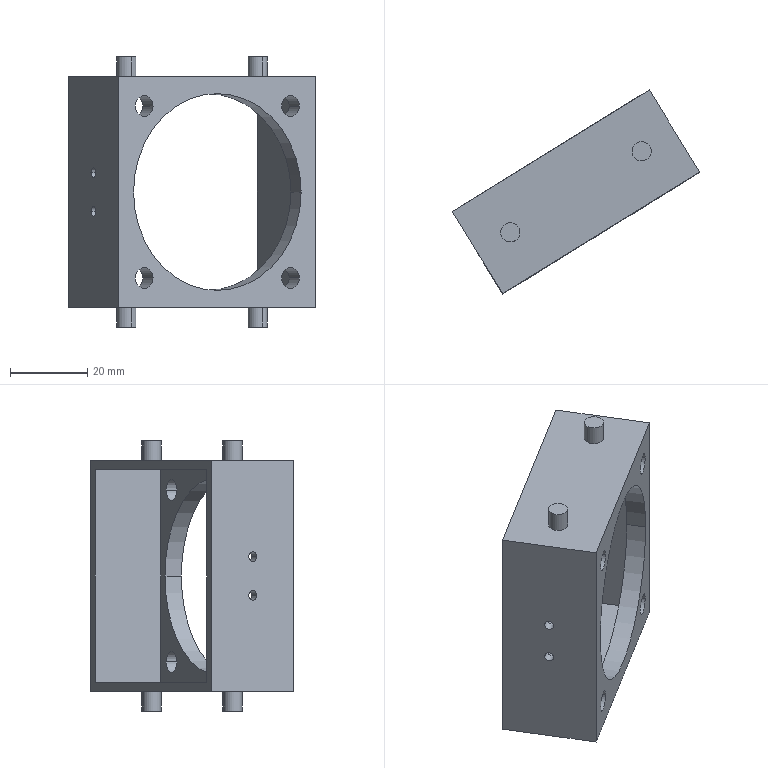Component | SolidWorks | WheelAssembly-1_MotorBracket-1 | 1 solid | 37 faces | box 64.19 x 52.78 x 70 mm | volume 19196 mm3 | cylinder 22 | plane 15 | commonest cylinder face diameters 5.4 x8 5 x8 2.5 x4 51 x2
build123d program:
from build123d import *

# Parameters (mm, degrees)
SKETCH1_W             = 60
SKETCH1_H             = 60
SKETCH1_R             = 25.5
BOSS_EXTRUDE1_DEPTH   = 5
SKETCH3_W             = 60
SKETCH3_H             = 60
SKETCH3_W_2           = 55
SKETCH3_H_2           = 55
BOSS_EXTRUDE2_DEPTH   = 20
SKETCH5_R             = 2.5
BOSS_EXTRUDE3_DEPTH   = 5
M3_TAPPED_HOLE1_D     = 2.5
M3_TAPPED_HOLE1_DEPTH = 7.5
M3_TAPPED_HOLE1_TIP   = 0.7511
SKETCH8_R             = 2.7
CUT_EXTRUDE1_DEPTH    = 30


with BuildPart() as part:
    # Sketch1 → Boss-Extrude1 (new body)
    with BuildSketch(Plane.XY):
        Rectangle(SKETCH1_W, SKETCH1_H)
        Circle(SKETCH1_R, mode=Mode.SUBTRACT)
    extrude(amount=BOSS_EXTRUDE1_DEPTH)

    # Sketch3 → Boss-Extrude2 (add)
    with BuildSketch(Plane(origin=(0, 0, 0), x_dir=(-1, 0, 0), z_dir=(0, 0, -1))):
        Rectangle(SKETCH3_W, SKETCH3_H)
        Rectangle(SKETCH3_W_2, SKETCH3_H_2, mode=Mode.SUBTRACT)
    extrude(amount=BOSS_EXTRUDE2_DEPTH)

    # Sketch5 → Boss-Extrude3 (add)
    with BuildSketch(Plane.XZ.offset(30)):
        with Locations(Location((-20, -7.5, 0), (0, 0, 90))):
            Circle(SKETCH5_R)
        with Locations(Location((20, -7.5, 0), (0, 0, 90))):
            Circle(SKETCH5_R)
    boss_extrude3 = extrude(amount=BOSS_EXTRUDE3_DEPTH)

    # Mirror1: Boss-Extrude3 across plane
    add(boss_extrude3.mirror(Plane.ZX))

    # M3 Tapped Hole1
    with Locations(Plane.ZY.offset(30)):
        with Locations((-7.5, 5), (-7.5, -5)):
            Hole(M3_TAPPED_HOLE1_D / 2, depth=M3_TAPPED_HOLE1_DEPTH)
            with Locations((0, 0, -(M3_TAPPED_HOLE1_DEPTH + M3_TAPPED_HOLE1_TIP / 2))):  # 118° drill point
                Cone(0, M3_TAPPED_HOLE1_D / 2, M3_TAPPED_HOLE1_TIP, mode=Mode.SUBTRACT)

    # Sketch8 → Cut-Extrude1 (cut)
    with BuildSketch(Plane.XY.offset(5)):
        with Locations((-22.274, 22.274)):
            Circle(SKETCH8_R)
        with Locations((22.274, 22.274)):
            Circle(SKETCH8_R)
        with Locations((22.274, -22.274)):
            Circle(SKETCH8_R)
        with Locations((-22.274, -22.274)):
            Circle(SKETCH8_R)
    extrude(amount=-CUT_EXTRUDE1_DEPTH, mode=Mode.SUBTRACT)


solid = part.part

# Placed as in the assembly
solid = solid.moved(Location((-217.384, -117.356, -542.97), (90, 31.668, 0)))